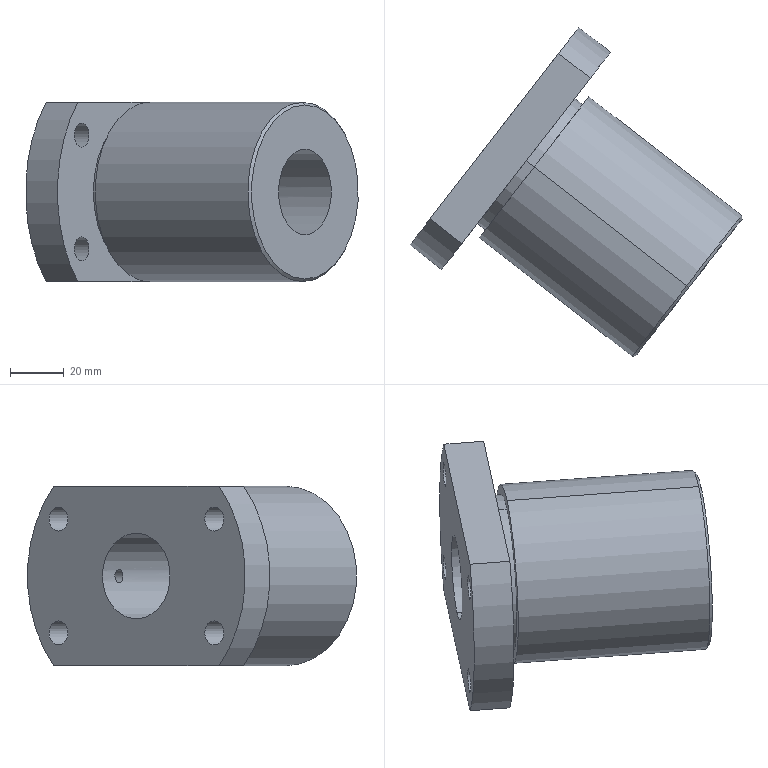Component | SolidWorks | MISUMI_BSSRK3210-800-F34-P20-1_NAT-2_MISUMI_BSSRK3210-800-F34-P20-1 | 1 solid | 26 faces | box 124.18 x 122.94 x 67 mm | volume 285610 mm3 | cylinder 18 | plane 6 | cone 2 | commonest cylinder face diameters 9 x8 4.917 x2 67 x2 59.3 x2 32 x2 103 x2
STEP:
#1=COLOUR_RGB('',0.7922,0.8196,0.9333);
#2=FILL_AREA_STYLE_COLOUR('',#1);
#3=FILL_AREA_STYLE('',(#2));
#4=SURFACE_STYLE_FILL_AREA(#3);
#5=SURFACE_SIDE_STYLE('',(#4));
#6=SURFACE_STYLE_USAGE(.BOTH.,#5);
#7=PRESENTATION_STYLE_ASSIGNMENT((#6));
#8=CARTESIAN_POINT('',(5.239,25.25,12.162));
#9=VERTEX_POINT('',#8);
#10=CARTESIAN_POINT('',(5.239,25.25,9.603));
#11=VERTEX_POINT('',#10);
#12=CARTESIAN_POINT('',(5.239,25.25,10.882));
#13=DIRECTION('',(0.7899,-0.6132,-0.));
#14=DIRECTION('',(0.,0.,-1.));
#15=AXIS2_PLACEMENT_3D('',#12,#13,#14);
#16=CIRCLE('',#15,1.28);
#17=EDGE_CURVE('',#9,#11,#16,.T.);
#18=ORIENTED_EDGE('',*,*,#17,.F.);
#19=CARTESIAN_POINT('',(5.208,25.274,12.201));
#20=VERTEX_POINT('',#19);
#21=CARTESIAN_POINT('',(5.239,25.25,12.162));
#22=DIRECTION('',(-0.5586,0.4336,0.7071));
#23=VECTOR('',#22,39.37);
#24=LINE('',#21,#23);
#25=EDGE_CURVE('',#9,#20,#24,.T.);
#26=ORIENTED_EDGE('',*,*,#25,.T.);
#27=CARTESIAN_POINT('',(5.208,25.274,9.563));
#28=VERTEX_POINT('',#27);
#29=CARTESIAN_POINT('',(5.208,25.274,10.882));
#30=DIRECTION('',(-0.7899,0.6132,0.));
#31=DIRECTION('',(0.,0.,-1.));
#32=AXIS2_PLACEMENT_3D('',#29,#30,#31);
#33=CIRCLE('',#32,1.319);
#34=EDGE_CURVE('',#28,#20,#33,.T.);
#35=ORIENTED_EDGE('',*,*,#34,.F.);
#36=CARTESIAN_POINT('',(5.239,25.25,9.603));
#37=DIRECTION('',(-0.5586,0.4336,-0.7071));
#38=VECTOR('',#37,39.37);
#39=LINE('',#36,#38);
#40=EDGE_CURVE('',#11,#28,#39,.T.);
#41=ORIENTED_EDGE('',*,*,#40,.F.);
#42=EDGE_LOOP('',(#18,#26,#35,#41));
#43=FACE_OUTER_BOUND('',#42,.T.);
#44=CARTESIAN_POINT('',(5.239,25.25,10.882));
#45=DIRECTION('',(-0.7899,0.6132,0.));
#46=DIRECTION('',(0.,0.,-1.));
#47=AXIS2_PLACEMENT_3D('',#44,#45,#46);
#48=CONICAL_SURFACE('',#47,1.28,0.7854);
#49=ADVANCED_FACE('',(#43),#48,.T.);
#50=CARTESIAN_POINT('',(3.071,27.721,10.979));
#51=VERTEX_POINT('',#50);
#52=CARTESIAN_POINT('',(3.071,27.721,10.786));
#53=VERTEX_POINT('',#52);
#54=CARTESIAN_POINT('',(3.071,27.721,10.979));
#55=CARTESIAN_POINT('',(3.081,27.713,10.979));
#56=CARTESIAN_POINT('',(3.091,27.706,10.977));
#57=CARTESIAN_POINT('',(3.105,27.696,10.969));
#58=CARTESIAN_POINT('',(3.11,27.693,10.966));
#59=CARTESIAN_POINT('',(3.119,27.687,10.959));
#60=CARTESIAN_POINT('',(3.123,27.684,10.955));
#61=CARTESIAN_POINT('',(3.131,27.68,10.946));
#62=CARTESIAN_POINT('',(3.134,27.677,10.941));
#63=CARTESIAN_POINT('',(3.14,27.674,10.931));
#64=CARTESIAN_POINT('',(3.143,27.672,10.925));
#65=CARTESIAN_POINT('',(3.147,27.67,10.914));
#66=CARTESIAN_POINT('',(3.149,27.669,10.907));
#67=CARTESIAN_POINT('',(3.151,27.668,10.895));
#68=CARTESIAN_POINT('',(3.152,27.667,10.889));
#69=CARTESIAN_POINT('',(3.152,27.667,10.876));
#70=CARTESIAN_POINT('',(3.151,27.668,10.87));
#71=CARTESIAN_POINT('',(3.149,27.669,10.857));
#72=CARTESIAN_POINT('',(3.147,27.67,10.851));
#73=CARTESIAN_POINT('',(3.143,27.672,10.839));
#74=CARTESIAN_POINT('',(3.141,27.674,10.834));
#75=CARTESIAN_POINT('',(3.134,27.677,10.823));
#76=CARTESIAN_POINT('',(3.131,27.68,10.818));
#77=CARTESIAN_POINT('',(3.119,27.687,10.805));
#78=CARTESIAN_POINT('',(3.11,27.692,10.798));
#79=CARTESIAN_POINT('',(3.096,27.702,10.791));
#80=CARTESIAN_POINT('',(3.091,27.706,10.789));
#81=CARTESIAN_POINT('',(3.081,27.713,10.786));
#82=CARTESIAN_POINT('',(3.076,27.717,10.786));
#83=CARTESIAN_POINT('',(3.071,27.721,10.786));
#84=B_SPLINE_CURVE_WITH_KNOTS('',3,(#54,#55,#56,#57,#58,#59,#60,#61,#62,#63,#64,#65,#66,#67,#68,#69,#70,#71,#72,#73,#74,#75,#76,#77,#78,#79,#80,#81,#82,#83),.UNSPECIFIED.,.F.,.F.,(4,2,2,2,2,2,2,2,2,2,2,2,2,2,4),(0.007698,0.00866,0.009141,0.009622,0.0101,0.01058,0.01106,0.01155,0.01203,0.01251,0.01299,0.01347,0.01443,0.01491,0.01539),.UNSPECIFIED.);
#85=EDGE_CURVE('',#51,#53,#84,.T.);
#86=ORIENTED_EDGE('',*,*,#85,.F.);
#87=CARTESIAN_POINT('',(3.931,28.829,10.979));
#88=VERTEX_POINT('',#87);
#89=CARTESIAN_POINT('',(3.932,28.831,10.979));
#90=DIRECTION('',(0.6132,0.7899,0.));
#91=VECTOR('',#90,39.37);
#92=LINE('',#89,#91);
#93=EDGE_CURVE('',#51,#88,#92,.T.);
#94=ORIENTED_EDGE('',*,*,#93,.T.);
#95=CARTESIAN_POINT('',(3.931,28.829,10.786));
#96=VERTEX_POINT('',#95);
#97=CARTESIAN_POINT('',(3.931,28.829,10.786));
#98=CARTESIAN_POINT('',(3.936,28.825,10.786));
#99=CARTESIAN_POINT('',(3.941,28.821,10.786));
#100=CARTESIAN_POINT('',(3.951,28.814,10.789));
#101=CARTESIAN_POINT('',(3.956,28.81,10.79));
#102=CARTESIAN_POINT('',(3.965,28.803,10.795));
#103=CARTESIAN_POINT('',(3.97,28.8,10.798));
#104=CARTESIAN_POINT('',(3.978,28.794,10.805));
#105=CARTESIAN_POINT('',(3.982,28.791,10.809));
#106=CARTESIAN_POINT('',(3.989,28.785,10.818));
#107=CARTESIAN_POINT('',(3.993,28.783,10.823));
#108=CARTESIAN_POINT('',(3.998,28.779,10.834));
#109=CARTESIAN_POINT('',(4.001,28.777,10.839));
#110=CARTESIAN_POINT('',(4.007,28.773,10.857));
#111=CARTESIAN_POINT('',(4.009,28.771,10.87));
#112=CARTESIAN_POINT('',(4.009,28.771,10.889));
#113=CARTESIAN_POINT('',(4.008,28.772,10.895));
#114=CARTESIAN_POINT('',(4.006,28.773,10.907));
#115=CARTESIAN_POINT('',(4.005,28.774,10.913));
#116=CARTESIAN_POINT('',(4.001,28.777,10.925));
#117=CARTESIAN_POINT('',(3.998,28.779,10.931));
#118=CARTESIAN_POINT('',(3.993,28.783,10.941));
#119=CARTESIAN_POINT('',(3.989,28.785,10.946));
#120=CARTESIAN_POINT('',(3.982,28.791,10.955));
#121=CARTESIAN_POINT('',(3.978,28.793,10.959));
#122=CARTESIAN_POINT('',(3.97,28.8,10.966));
#123=CARTESIAN_POINT('',(3.965,28.803,10.969));
#124=CARTESIAN_POINT('',(3.956,28.81,10.974));
#125=CARTESIAN_POINT('',(3.951,28.814,10.976));
#126=CARTESIAN_POINT('',(3.941,28.821,10.978));
#127=CARTESIAN_POINT('',(3.936,28.825,10.979));
#128=CARTESIAN_POINT('',(3.931,28.829,10.979));
#129=B_SPLINE_CURVE_WITH_KNOTS('',3,(#97,#98,#99,#100,#101,#102,#103,#104,#105,#106,#107,#108,#109,#110,#111,#112,#113,#114,#115,#116,#117,#118,#119,#120,#121,#122,#123,#124,#125,#126,#127,#128),.UNSPECIFIED.,.F.,.F.,(4,2,2,2,2,2,2,2,2,2,2,2,2,2,2,4),(0.,0.0004805,0.0009609,0.001441,0.001922,0.002402,0.002883,0.003844,0.004324,0.004805,0.005285,0.005766,0.006246,0.006727,0.007207,0.007687),.UNSPECIFIED.);
#130=EDGE_CURVE('',#96,#88,#129,.T.);
#131=ORIENTED_EDGE('',*,*,#130,.F.);
#132=CARTESIAN_POINT('',(3.932,28.831,10.786));
#133=DIRECTION('',(0.6132,0.7899,0.));
#134=VECTOR('',#133,39.37);
#135=LINE('',#132,#134);
#136=EDGE_CURVE('',#53,#96,#135,.T.);
#137=ORIENTED_EDGE('',*,*,#136,.F.);
#138=EDGE_LOOP('',(#86,#94,#131,#137));
#139=FACE_OUTER_BOUND('',#138,.T.);
#140=CARTESIAN_POINT('',(3.932,28.831,10.882));
#141=DIRECTION('',(0.6132,0.7899,0.));
#142=DIRECTION('',(0.,0.,-1.));
#143=AXIS2_PLACEMENT_3D('',#140,#141,#142);
#144=CYLINDRICAL_SURFACE('',#143,0.09679);
#145=ADVANCED_FACE('',(#139),#144,.F.);
#146=CARTESIAN_POINT('',(3.267,28.615,10.223));
#147=VERTEX_POINT('',#146);
#148=CARTESIAN_POINT('',(3.267,28.615,9.869));
#149=VERTEX_POINT('',#148);
#150=CARTESIAN_POINT('',(3.267,28.615,10.046));
#151=DIRECTION('',(-0.7899,0.6132,0.));
#152=DIRECTION('',(0.,0.,-1.));
#153=AXIS2_PLACEMENT_3D('',#150,#151,#152);
#154=CIRCLE('',#153,0.1772);
#155=EDGE_CURVE('',#147,#149,#154,.T.);
#156=ORIENTED_EDGE('',*,*,#155,.T.);
#157=CARTESIAN_POINT('',(3.733,28.253,9.869));
#158=VERTEX_POINT('',#157);
#159=CARTESIAN_POINT('',(3.267,28.615,9.869));
#160=DIRECTION('',(0.7899,-0.6132,-0.));
#161=VECTOR('',#160,39.37);
#162=LINE('',#159,#161);
#163=EDGE_CURVE('',#149,#158,#162,.T.);
#164=ORIENTED_EDGE('',*,*,#163,.T.);
#165=CARTESIAN_POINT('',(3.733,28.253,10.223));
#166=VERTEX_POINT('',#165);
#167=CARTESIAN_POINT('',(3.733,28.253,10.046));
#168=DIRECTION('',(-0.7899,0.6132,0.));
#169=DIRECTION('',(0.,0.,-1.));
#170=AXIS2_PLACEMENT_3D('',#167,#168,#169);
#171=CIRCLE('',#170,0.1772);
#172=EDGE_CURVE('',#166,#158,#171,.T.);
#173=ORIENTED_EDGE('',*,*,#172,.F.);
#174=CARTESIAN_POINT('',(3.267,28.615,10.223));
#175=DIRECTION('',(0.7899,-0.6132,-0.));
#176=VECTOR('',#175,39.37);
#177=LINE('',#174,#176);
#178=EDGE_CURVE('',#147,#166,#177,.T.);
#179=ORIENTED_EDGE('',*,*,#178,.F.);
#180=EDGE_LOOP('',(#156,#164,#173,#179));
#181=FACE_OUTER_BOUND('',#180,.T.);
#182=CARTESIAN_POINT('',(3.267,28.615,10.046));
#183=DIRECTION('',(0.7899,-0.6132,-0.));
#184=DIRECTION('',(-0.,-0.,1.));
#185=AXIS2_PLACEMENT_3D('',#182,#183,#184);
#186=CYLINDRICAL_SURFACE('',#185,0.1772);
#187=ADVANCED_FACE('',(#181),#186,.F.);
#188=CARTESIAN_POINT('',(3.267,28.615,11.896));
#189=VERTEX_POINT('',#188);
#190=CARTESIAN_POINT('',(3.267,28.615,11.542));
#191=VERTEX_POINT('',#190);
#192=CARTESIAN_POINT('',(3.267,28.615,11.719));
#193=DIRECTION('',(-0.7899,0.6132,0.));
#194=DIRECTION('',(0.,0.,-1.));
#195=AXIS2_PLACEMENT_3D('',#192,#193,#194);
#196=CIRCLE('',#195,0.1772);
#197=EDGE_CURVE('',#189,#191,#196,.T.);
#198=ORIENTED_EDGE('',*,*,#197,.T.);
#199=CARTESIAN_POINT('',(3.733,28.253,11.542));
#200=VERTEX_POINT('',#199);
#201=CARTESIAN_POINT('',(3.267,28.615,11.542));
#202=DIRECTION('',(0.7899,-0.6132,-0.));
#203=VECTOR('',#202,39.37);
#204=LINE('',#201,#203);
#205=EDGE_CURVE('',#191,#200,#204,.T.);
#206=ORIENTED_EDGE('',*,*,#205,.T.);
#207=CARTESIAN_POINT('',(3.733,28.253,11.896));
#208=VERTEX_POINT('',#207);
#209=CARTESIAN_POINT('',(3.733,28.253,11.719));
#210=DIRECTION('',(-0.7899,0.6132,0.));
#211=DIRECTION('',(0.,0.,-1.));
#212=AXIS2_PLACEMENT_3D('',#209,#210,#211);
#213=CIRCLE('',#212,0.1772);
#214=EDGE_CURVE('',#208,#200,#213,.T.);
#215=ORIENTED_EDGE('',*,*,#214,.F.);
#216=CARTESIAN_POINT('',(3.267,28.615,11.896));
#217=DIRECTION('',(0.7899,-0.6132,-0.));
#218=VECTOR('',#217,39.37);
#219=LINE('',#216,#218);
#220=EDGE_CURVE('',#189,#208,#219,.T.);
#221=ORIENTED_EDGE('',*,*,#220,.F.);
#222=EDGE_LOOP('',(#198,#206,#215,#221));
#223=FACE_OUTER_BOUND('',#222,.T.);
#224=CARTESIAN_POINT('',(3.267,28.615,11.719));
#225=DIRECTION('',(0.7899,-0.6132,-0.));
#226=DIRECTION('',(-0.,-0.,1.));
#227=AXIS2_PLACEMENT_3D('',#224,#225,#226);
#228=CYLINDRICAL_SURFACE('',#227,0.1772);
#229=ADVANCED_FACE('',(#223),#228,.F.);
#230=CARTESIAN_POINT('',(1.489,26.326,11.896));
#231=VERTEX_POINT('',#230);
#232=CARTESIAN_POINT('',(1.489,26.326,11.542));
#233=VERTEX_POINT('',#232);
#234=CARTESIAN_POINT('',(1.489,26.326,11.719));
#235=DIRECTION('',(-0.7899,0.6132,0.));
#236=DIRECTION('',(0.,0.,-1.));
#237=AXIS2_PLACEMENT_3D('',#234,#235,#236);
#238=CIRCLE('',#237,0.1772);
#239=EDGE_CURVE('',#231,#233,#238,.T.);
#240=ORIENTED_EDGE('',*,*,#239,.T.);
#241=CARTESIAN_POINT('',(1.956,25.964,11.542));
#242=VERTEX_POINT('',#241);
#243=CARTESIAN_POINT('',(1.489,26.326,11.542));
#244=DIRECTION('',(0.7899,-0.6132,-0.));
#245=VECTOR('',#244,39.37);
#246=LINE('',#243,#245);
#247=EDGE_CURVE('',#233,#242,#246,.T.);
#248=ORIENTED_EDGE('',*,*,#247,.T.);
#249=CARTESIAN_POINT('',(1.956,25.964,11.896));
#250=VERTEX_POINT('',#249);
#251=CARTESIAN_POINT('',(1.956,25.964,11.719));
#252=DIRECTION('',(-0.7899,0.6132,0.));
#253=DIRECTION('',(0.,0.,-1.));
#254=AXIS2_PLACEMENT_3D('',#251,#252,#253);
#255=CIRCLE('',#254,0.1772);
#256=EDGE_CURVE('',#250,#242,#255,.T.);
#257=ORIENTED_EDGE('',*,*,#256,.F.);
#258=CARTESIAN_POINT('',(1.489,26.326,11.896));
#259=DIRECTION('',(0.7899,-0.6132,-0.));
#260=VECTOR('',#259,39.37);
#261=LINE('',#258,#260);
#262=EDGE_CURVE('',#231,#250,#261,.T.);
#263=ORIENTED_EDGE('',*,*,#262,.F.);
#264=EDGE_LOOP('',(#240,#248,#257,#263));
#265=FACE_OUTER_BOUND('',#264,.T.);
#266=CARTESIAN_POINT('',(1.489,26.326,11.719));
#267=DIRECTION('',(0.7899,-0.6132,-0.));
#268=DIRECTION('',(-0.,-0.,1.));
#269=AXIS2_PLACEMENT_3D('',#266,#267,#268);
#270=CYLINDRICAL_SURFACE('',#269,0.1772);
#271=ADVANCED_FACE('',(#265),#270,.F.);
#272=CARTESIAN_POINT('',(1.489,26.326,10.223));
#273=VERTEX_POINT('',#272);
#274=CARTESIAN_POINT('',(1.489,26.326,9.869));
#275=VERTEX_POINT('',#274);
#276=CARTESIAN_POINT('',(1.489,26.326,10.046));
#277=DIRECTION('',(-0.7899,0.6132,0.));
#278=DIRECTION('',(0.,0.,-1.));
#279=AXIS2_PLACEMENT_3D('',#276,#277,#278);
#280=CIRCLE('',#279,0.1772);
#281=EDGE_CURVE('',#273,#275,#280,.T.);
#282=ORIENTED_EDGE('',*,*,#281,.T.);
#283=CARTESIAN_POINT('',(1.956,25.964,9.869));
#284=VERTEX_POINT('',#283);
#285=CARTESIAN_POINT('',(1.489,26.326,9.869));
#286=DIRECTION('',(0.7899,-0.6132,-0.));
#287=VECTOR('',#286,39.37);
#288=LINE('',#285,#287);
#289=EDGE_CURVE('',#275,#284,#288,.T.);
#290=ORIENTED_EDGE('',*,*,#289,.T.);
#291=CARTESIAN_POINT('',(1.956,25.964,10.223));
#292=VERTEX_POINT('',#291);
#293=CARTESIAN_POINT('',(1.956,25.964,10.046));
#294=DIRECTION('',(-0.7899,0.6132,0.));
#295=DIRECTION('',(0.,0.,-1.));
#296=AXIS2_PLACEMENT_3D('',#293,#294,#295);
#297=CIRCLE('',#296,0.1772);
#298=EDGE_CURVE('',#292,#284,#297,.T.);
#299=ORIENTED_EDGE('',*,*,#298,.F.);
#300=CARTESIAN_POINT('',(1.489,26.326,10.223));
#301=DIRECTION('',(0.7899,-0.6132,-0.));
#302=VECTOR('',#301,39.37);
#303=LINE('',#300,#302);
#304=EDGE_CURVE('',#273,#292,#303,.T.);
#305=ORIENTED_EDGE('',*,*,#304,.F.);
#306=EDGE_LOOP('',(#282,#290,#299,#305));
#307=FACE_OUTER_BOUND('',#306,.T.);
#308=CARTESIAN_POINT('',(1.489,26.326,10.046));
#309=DIRECTION('',(0.7899,-0.6132,-0.));
#310=DIRECTION('',(-0.,-0.,1.));
#311=AXIS2_PLACEMENT_3D('',#308,#309,#310);
#312=CYLINDRICAL_SURFACE('',#311,0.1772);
#313=ADVANCED_FACE('',(#307),#312,.F.);
#314=CARTESIAN_POINT('',(2.964,27.016,12.201));
#315=VERTEX_POINT('',#314);
#316=CARTESIAN_POINT('',(2.964,27.016,9.563));
#317=VERTEX_POINT('',#316);
#318=CARTESIAN_POINT('',(2.964,27.016,10.882));
#319=DIRECTION('',(0.7899,-0.6132,-0.));
#320=DIRECTION('',(-0.,-0.,1.));
#321=AXIS2_PLACEMENT_3D('',#318,#319,#320);
#322=CIRCLE('',#321,1.319);
#323=EDGE_CURVE('',#315,#317,#322,.T.);
#324=ORIENTED_EDGE('',*,*,#323,.T.);
#325=CARTESIAN_POINT('',(5.239,25.25,9.563));
#326=DIRECTION('',(0.7899,-0.6132,-0.));
#327=VECTOR('',#326,39.37);
#328=LINE('',#325,#327);
#329=EDGE_CURVE('',#317,#28,#328,.T.);
#330=ORIENTED_EDGE('',*,*,#329,.T.);
#331=ORIENTED_EDGE('',*,*,#34,.T.);
#332=CARTESIAN_POINT('',(5.239,25.25,12.201));
#333=DIRECTION('',(0.7899,-0.6132,-0.));
#334=VECTOR('',#333,39.37);
#335=LINE('',#332,#334);
#336=EDGE_CURVE('',#315,#20,#335,.T.);
#337=ORIENTED_EDGE('',*,*,#336,.F.);
#338=EDGE_LOOP('',(#324,#330,#331,#337));
#339=FACE_OUTER_BOUND('',#338,.T.);
#340=CARTESIAN_POINT('',(5.239,25.25,10.882));
#341=DIRECTION('',(0.7899,-0.6132,-0.));
#342=DIRECTION('',(-0.,-0.,1.));
#343=AXIS2_PLACEMENT_3D('',#340,#341,#342);
#344=CYLINDRICAL_SURFACE('',#343,1.319);
#345=ADVANCED_FACE('',(#339),#344,.T.);
#346=CARTESIAN_POINT('',(2.844,27.108,12.05));
#347=VERTEX_POINT('',#346);
#348=CARTESIAN_POINT('',(2.844,27.108,9.715));
#349=VERTEX_POINT('',#348);
#350=CARTESIAN_POINT('',(2.844,27.108,10.882));
#351=DIRECTION('',(0.7899,-0.6132,-0.));
#352=DIRECTION('',(-0.,-0.,1.));
#353=AXIS2_PLACEMENT_3D('',#350,#351,#352);
#354=CIRCLE('',#353,1.167);
#355=EDGE_CURVE('',#347,#349,#354,.T.);
#356=ORIENTED_EDGE('',*,*,#355,.T.);
#357=CARTESIAN_POINT('',(2.964,27.016,9.715));
#358=VERTEX_POINT('',#357);
#359=CARTESIAN_POINT('',(5.239,25.25,9.715));
#360=DIRECTION('',(0.7899,-0.6132,-0.));
#361=VECTOR('',#360,39.37);
#362=LINE('',#359,#361);
#363=EDGE_CURVE('',#349,#358,#362,.T.);
#364=ORIENTED_EDGE('',*,*,#363,.T.);
#365=CARTESIAN_POINT('',(2.964,27.016,12.05));
#366=VERTEX_POINT('',#365);
#367=CARTESIAN_POINT('',(2.964,27.016,10.882));
#368=DIRECTION('',(0.7899,-0.6132,-0.));
#369=DIRECTION('',(-0.,-0.,1.));
#370=AXIS2_PLACEMENT_3D('',#367,#368,#369);
#371=CIRCLE('',#370,1.167);
#372=EDGE_CURVE('',#366,#358,#371,.T.);
#373=ORIENTED_EDGE('',*,*,#372,.F.);
#374=CARTESIAN_POINT('',(5.239,25.25,12.05));
#375=DIRECTION('',(0.7899,-0.6132,-0.));
#376=VECTOR('',#375,39.37);
#377=LINE('',#374,#376);
#378=EDGE_CURVE('',#347,#366,#377,.T.);
#379=ORIENTED_EDGE('',*,*,#378,.F.);
#380=EDGE_LOOP('',(#356,#364,#373,#379));
#381=FACE_OUTER_BOUND('',#380,.T.);
#382=CARTESIAN_POINT('',(5.239,25.25,10.882));
#383=DIRECTION('',(0.7899,-0.6132,-0.));
#384=DIRECTION('',(-0.,-0.,1.));
#385=AXIS2_PLACEMENT_3D('',#382,#383,#384);
#386=CYLINDRICAL_SURFACE('',#385,1.167);
#387=ADVANCED_FACE('',(#381),#386,.T.);
#388=CARTESIAN_POINT('',(3.071,27.721,10.786));
#389=CARTESIAN_POINT('',(3.066,27.725,10.786));
#390=CARTESIAN_POINT('',(3.061,27.729,10.786));
#391=CARTESIAN_POINT('',(3.051,27.737,10.789));
#392=CARTESIAN_POINT('',(3.046,27.741,10.79));
#393=CARTESIAN_POINT('',(3.038,27.748,10.795));
#394=CARTESIAN_POINT('',(3.033,27.752,10.798));
#395=CARTESIAN_POINT('',(3.026,27.759,10.805));
#396=CARTESIAN_POINT('',(3.022,27.763,10.809));
#397=CARTESIAN_POINT('',(3.012,27.772,10.823));
#398=CARTESIAN_POINT('',(3.007,27.777,10.834));
#399=CARTESIAN_POINT('',(3.002,27.783,10.851));
#400=CARTESIAN_POINT('',(3.001,27.784,10.857));
#401=CARTESIAN_POINT('',(2.999,27.786,10.87));
#402=CARTESIAN_POINT('',(2.999,27.786,10.876));
#403=CARTESIAN_POINT('',(2.999,27.786,10.889));
#404=CARTESIAN_POINT('',(2.999,27.786,10.895));
#405=CARTESIAN_POINT('',(3.001,27.784,10.907));
#406=CARTESIAN_POINT('',(3.002,27.783,10.914));
#407=CARTESIAN_POINT('',(3.006,27.779,10.925));
#408=CARTESIAN_POINT('',(3.008,27.777,10.931));
#409=CARTESIAN_POINT('',(3.013,27.772,10.941));
#410=CARTESIAN_POINT('',(3.016,27.769,10.946));
#411=CARTESIAN_POINT('',(3.022,27.763,10.955));
#412=CARTESIAN_POINT('',(3.026,27.759,10.959));
#413=CARTESIAN_POINT('',(3.033,27.752,10.966));
#414=CARTESIAN_POINT('',(3.038,27.748,10.969));
#415=CARTESIAN_POINT('',(3.046,27.741,10.974));
#416=CARTESIAN_POINT('',(3.051,27.737,10.976));
#417=CARTESIAN_POINT('',(3.061,27.729,10.978));
#418=CARTESIAN_POINT('',(3.066,27.725,10.979));
#419=CARTESIAN_POINT('',(3.071,27.721,10.979));
#420=B_SPLINE_CURVE_WITH_KNOTS('',3,(#388,#389,#390,#391,#392,#393,#394,#395,#396,#397,#398,#399,#400,#401,#402,#403,#404,#405,#406,#407,#408,#409,#410,#411,#412,#413,#414,#415,#416,#417,#418,#419),.UNSPECIFIED.,.F.,.F.,(4,2,2,2,2,2,2,2,2,2,2,2,2,2,2,4),(0.,0.0004811,0.0009622,0.001443,0.001924,0.002887,0.003368,0.003849,0.00433,0.004811,0.005292,0.005773,0.006254,0.006736,0.007217,0.007698),.UNSPECIFIED.);
#421=EDGE_CURVE('',#53,#51,#420,.T.);
#422=ORIENTED_EDGE('',*,*,#421,.T.);
#423=ORIENTED_EDGE('',*,*,#85,.T.);
#424=EDGE_LOOP('',(#422,#423));
#425=FACE_BOUND('',#424,.T.);
#426=CARTESIAN_POINT('',(2.378,27.471,10.252));
#427=VERTEX_POINT('',#426);
#428=CARTESIAN_POINT('',(2.378,27.471,11.512));
#429=VERTEX_POINT('',#428);
#430=CARTESIAN_POINT('',(2.378,27.471,10.882));
#431=DIRECTION('',(0.7899,-0.6132,-0.));
#432=DIRECTION('',(-0.,-0.,1.));
#433=AXIS2_PLACEMENT_3D('',#430,#431,#432);
#434=CIRCLE('',#433,0.6299);
#435=EDGE_CURVE('',#427,#429,#434,.T.);
#436=ORIENTED_EDGE('',*,*,#435,.F.);
#437=CARTESIAN_POINT('',(5.239,25.25,10.252));
#438=VERTEX_POINT('',#437);
#439=CARTESIAN_POINT('',(5.239,25.25,10.252));
#440=DIRECTION('',(0.7899,-0.6132,-0.));
#441=VECTOR('',#440,39.37);
#442=LINE('',#439,#441);
#443=EDGE_CURVE('',#427,#438,#442,.T.);
#444=ORIENTED_EDGE('',*,*,#443,.T.);
#445=CARTESIAN_POINT('',(5.239,25.25,11.512));
#446=VERTEX_POINT('',#445);
#447=CARTESIAN_POINT('',(5.239,25.25,10.882));
#448=DIRECTION('',(0.7899,-0.6132,-0.));
#449=DIRECTION('',(-0.,-0.,1.));
#450=AXIS2_PLACEMENT_3D('',#447,#448,#449);
#451=CIRCLE('',#450,0.6299);
#452=EDGE_CURVE('',#438,#446,#451,.T.);
#453=ORIENTED_EDGE('',*,*,#452,.T.);
#454=CARTESIAN_POINT('',(5.239,25.25,11.512));
#455=DIRECTION('',(0.7899,-0.6132,-0.));
#456=VECTOR('',#455,39.37);
#457=LINE('',#454,#456);
#458=EDGE_CURVE('',#429,#446,#457,.T.);
#459=ORIENTED_EDGE('',*,*,#458,.F.);
#460=EDGE_LOOP('',(#436,#444,#453,#459));
#461=FACE_OUTER_BOUND('',#460,.T.);
#462=CARTESIAN_POINT('',(5.239,25.25,10.882));
#463=DIRECTION('',(0.7899,-0.6132,-0.));
#464=DIRECTION('',(-0.,-0.,1.));
#465=AXIS2_PLACEMENT_3D('',#462,#463,#464);
#466=CYLINDRICAL_SURFACE('',#465,0.6299);
#467=ADVANCED_FACE('',(#425,#461),#466,.F.);
#468=CARTESIAN_POINT('',(2.378,27.471,10.882));
#469=DIRECTION('',(0.7899,-0.6132,-0.));
#470=DIRECTION('',(-0.,-0.,1.));
#471=AXIS2_PLACEMENT_3D('',#468,#469,#470);
#472=CIRCLE('',#471,0.6299);
#473=EDGE_CURVE('',#429,#427,#472,.T.);
#474=ORIENTED_EDGE('',*,*,#473,.T.);
#475=ORIENTED_EDGE('',*,*,#435,.T.);
#476=EDGE_LOOP('',(#474,#475));
#477=FACE_BOUND('',#476,.T.);
#478=CARTESIAN_POINT('',(3.322,28.687,12.201));
#479=VERTEX_POINT('',#478);
#480=CARTESIAN_POINT('',(1.434,26.254,12.201));
#481=VERTEX_POINT('',#480);
#482=CARTESIAN_POINT('',(1.434,26.254,12.201));
#483=DIRECTION('',(-0.6132,-0.7899,-0.));
#484=VECTOR('',#483,39.37);
#485=LINE('',#482,#484);
#486=EDGE_CURVE('',#479,#481,#485,.T.);
#487=ORIENTED_EDGE('',*,*,#486,.F.);
#488=CARTESIAN_POINT('',(3.322,28.687,9.563));
#489=VERTEX_POINT('',#488);
#490=CARTESIAN_POINT('',(2.378,27.471,10.882));
#491=DIRECTION('',(0.7899,-0.6132,-0.));
#492=DIRECTION('',(-0.,-0.,1.));
#493=AXIS2_PLACEMENT_3D('',#490,#491,#492);
#494=CIRCLE('',#493,2.028);
#495=EDGE_CURVE('',#489,#479,#494,.T.);
#496=ORIENTED_EDGE('',*,*,#495,.F.);
#497=CARTESIAN_POINT('',(1.434,26.254,9.563));
#498=VERTEX_POINT('',#497);
#499=CARTESIAN_POINT('',(1.434,26.254,9.563));
#500=DIRECTION('',(0.6132,0.7899,0.));
#501=VECTOR('',#500,39.37);
#502=LINE('',#499,#501);
#503=EDGE_CURVE('',#498,#489,#502,.T.);
#504=ORIENTED_EDGE('',*,*,#503,.F.);
#505=CARTESIAN_POINT('',(2.378,27.471,10.882));
#506=DIRECTION('',(0.7899,-0.6132,-0.));
#507=DIRECTION('',(-0.,-0.,1.));
#508=AXIS2_PLACEMENT_3D('',#505,#506,#507);
#509=CIRCLE('',#508,2.028);
#510=EDGE_CURVE('',#481,#498,#509,.T.);
#511=ORIENTED_EDGE('',*,*,#510,.F.);
#512=EDGE_LOOP('',(#487,#496,#504,#511));
#513=FACE_OUTER_BOUND('',#512,.T.);
#514=ORIENTED_EDGE('',*,*,#281,.F.);
#515=CARTESIAN_POINT('',(1.489,26.326,10.046));
#516=DIRECTION('',(-0.7899,0.6132,0.));
#517=DIRECTION('',(0.,0.,-1.));
#518=AXIS2_PLACEMENT_3D('',#515,#516,#517);
#519=CIRCLE('',#518,0.1772);
#520=EDGE_CURVE('',#275,#273,#519,.T.);
#521=ORIENTED_EDGE('',*,*,#520,.F.);
#522=EDGE_LOOP('',(#514,#521));
#523=FACE_BOUND('',#522,.T.);
#524=ORIENTED_EDGE('',*,*,#239,.F.);
#525=CARTESIAN_POINT('',(1.489,26.326,11.719));
#526=DIRECTION('',(-0.7899,0.6132,0.));
#527=DIRECTION('',(0.,0.,-1.));
#528=AXIS2_PLACEMENT_3D('',#525,#526,#527);
#529=CIRCLE('',#528,0.1772);
#530=EDGE_CURVE('',#233,#231,#529,.T.);
#531=ORIENTED_EDGE('',*,*,#530,.F.);
#532=EDGE_LOOP('',(#524,#531));
#533=FACE_BOUND('',#532,.T.);
#534=ORIENTED_EDGE('',*,*,#197,.F.);
#535=CARTESIAN_POINT('',(3.267,28.615,11.719));
#536=DIRECTION('',(-0.7899,0.6132,0.));
#537=DIRECTION('',(0.,0.,-1.));
#538=AXIS2_PLACEMENT_3D('',#535,#536,#537);
#539=CIRCLE('',#538,0.1772);
#540=EDGE_CURVE('',#191,#189,#539,.T.);
#541=ORIENTED_EDGE('',*,*,#540,.F.);
#542=EDGE_LOOP('',(#534,#541));
#543=FACE_BOUND('',#542,.T.);
#544=ORIENTED_EDGE('',*,*,#155,.F.);
#545=CARTESIAN_POINT('',(3.267,28.615,10.046));
#546=DIRECTION('',(-0.7899,0.6132,0.));
#547=DIRECTION('',(0.,0.,-1.));
#548=AXIS2_PLACEMENT_3D('',#545,#546,#547);
#549=CIRCLE('',#548,0.1772);
#550=EDGE_CURVE('',#149,#147,#549,.T.);
#551=ORIENTED_EDGE('',*,*,#550,.F.);
#552=EDGE_LOOP('',(#544,#551));
#553=FACE_BOUND('',#552,.T.);
#554=CARTESIAN_POINT('',(1.992,26.973,10.882));
#555=DIRECTION('',(0.7899,-0.6132,-0.));
#556=DIRECTION('',(-0.,-0.,1.));
#557=AXIS2_PLACEMENT_3D('',#554,#555,#556);
#558=PLANE('',#557);
#559=ADVANCED_FACE('',(#477,#513,#523,#533,#543,#553),#558,.F.);
#560=ORIENTED_EDGE('',*,*,#355,.F.);
#561=CARTESIAN_POINT('',(2.844,27.108,10.882));
#562=DIRECTION('',(0.7899,-0.6132,-0.));
#563=DIRECTION('',(-0.,-0.,1.));
#564=AXIS2_PLACEMENT_3D('',#561,#562,#563);
#565=CIRCLE('',#564,1.167);
#566=EDGE_CURVE('',#349,#347,#565,.T.);
#567=ORIENTED_EDGE('',*,*,#566,.F.);
#568=EDGE_LOOP('',(#560,#567));
#569=FACE_BOUND('',#568,.T.);
#570=CARTESIAN_POINT('',(3.789,28.325,12.201));
#571=VERTEX_POINT('',#570);
#572=CARTESIAN_POINT('',(1.9,25.892,12.201));
#573=VERTEX_POINT('',#572);
#574=CARTESIAN_POINT('',(1.9,25.892,12.201));
#575=DIRECTION('',(-0.6132,-0.7899,-0.));
#576=VECTOR('',#575,39.37);
#577=LINE('',#574,#576);
#578=EDGE_CURVE('',#571,#573,#577,.T.);
#579=ORIENTED_EDGE('',*,*,#578,.T.);
#580=CARTESIAN_POINT('',(1.9,25.892,9.563));
#581=VERTEX_POINT('',#580);
#582=CARTESIAN_POINT('',(2.844,27.108,10.882));
#583=DIRECTION('',(0.7899,-0.6132,-0.));
#584=DIRECTION('',(-0.,-0.,1.));
#585=AXIS2_PLACEMENT_3D('',#582,#583,#584);
#586=CIRCLE('',#585,2.028);
#587=EDGE_CURVE('',#573,#581,#586,.T.);
#588=ORIENTED_EDGE('',*,*,#587,.T.);
#589=CARTESIAN_POINT('',(3.789,28.325,9.563));
#590=VERTEX_POINT('',#589);
#591=CARTESIAN_POINT('',(1.9,25.892,9.563));
#592=DIRECTION('',(0.6132,0.7899,0.));
#593=VECTOR('',#592,39.37);
#594=LINE('',#591,#593);
#595=EDGE_CURVE('',#581,#590,#594,.T.);
#596=ORIENTED_EDGE('',*,*,#595,.T.);
#597=CARTESIAN_POINT('',(2.844,27.108,10.882));
#598=DIRECTION('',(0.7899,-0.6132,-0.));
#599=DIRECTION('',(-0.,-0.,1.));
#600=AXIS2_PLACEMENT_3D('',#597,#598,#599);
#601=CIRCLE('',#600,2.028);
#602=EDGE_CURVE('',#590,#571,#601,.T.);
#603=ORIENTED_EDGE('',*,*,#602,.T.);
#604=EDGE_LOOP('',(#579,#588,#596,#603));
#605=FACE_OUTER_BOUND('',#604,.T.);
#606=ORIENTED_EDGE('',*,*,#298,.T.);
#607=CARTESIAN_POINT('',(1.956,25.964,10.046));
#608=DIRECTION('',(-0.7899,0.6132,0.));
#609=DIRECTION('',(0.,0.,-1.));
#610=AXIS2_PLACEMENT_3D('',#607,#608,#609);
#611=CIRCLE('',#610,0.1772);
#612=EDGE_CURVE('',#284,#292,#611,.T.);
#613=ORIENTED_EDGE('',*,*,#612,.T.);
#614=EDGE_LOOP('',(#606,#613));
#615=FACE_BOUND('',#614,.T.);
#616=ORIENTED_EDGE('',*,*,#256,.T.);
#617=CARTESIAN_POINT('',(1.956,25.964,11.719));
#618=DIRECTION('',(-0.7899,0.6132,0.));
#619=DIRECTION('',(0.,0.,-1.));
#620=AXIS2_PLACEMENT_3D('',#617,#618,#619);
#621=CIRCLE('',#620,0.1772);
#622=EDGE_CURVE('',#242,#250,#621,.T.);
#623=ORIENTED_EDGE('',*,*,#622,.T.);
#624=EDGE_LOOP('',(#616,#623));
#625=FACE_BOUND('',#624,.T.);
#626=ORIENTED_EDGE('',*,*,#214,.T.);
#627=CARTESIAN_POINT('',(3.733,28.253,11.719));
#628=DIRECTION('',(-0.7899,0.6132,0.));
#629=DIRECTION('',(0.,0.,-1.));
#630=AXIS2_PLACEMENT_3D('',#627,#628,#629);
#631=CIRCLE('',#630,0.1772);
#632=EDGE_CURVE('',#200,#208,#631,.T.);
#633=ORIENTED_EDGE('',*,*,#632,.T.);
#634=EDGE_LOOP('',(#626,#633));
#635=FACE_BOUND('',#634,.T.);
#636=ORIENTED_EDGE('',*,*,#172,.T.);
#637=CARTESIAN_POINT('',(3.733,28.253,10.046));
#638=DIRECTION('',(-0.7899,0.6132,0.));
#639=DIRECTION('',(0.,0.,-1.));
#640=AXIS2_PLACEMENT_3D('',#637,#638,#639);
#641=CIRCLE('',#640,0.1772);
#642=EDGE_CURVE('',#158,#166,#641,.T.);
#643=ORIENTED_EDGE('',*,*,#642,.T.);
#644=EDGE_LOOP('',(#636,#643));
#645=FACE_BOUND('',#644,.T.);
#646=CARTESIAN_POINT('',(1.601,25.507,10.882));
#647=DIRECTION('',(-0.7899,0.6132,0.));
#648=DIRECTION('',(0.,0.,-1.));
#649=AXIS2_PLACEMENT_3D('',#646,#647,#648);
#650=PLANE('',#649);
#651=ADVANCED_FACE('',(#569,#605,#615,#625,#635,#645),#650,.F.);
#652=CARTESIAN_POINT('',(1.434,26.254,12.201));
#653=DIRECTION('',(0.7899,-0.6132,-0.));
#654=VECTOR('',#653,39.37);
#655=LINE('',#652,#654);
#656=EDGE_CURVE('',#481,#573,#655,.T.);
#657=ORIENTED_EDGE('',*,*,#656,.F.);
#658=ORIENTED_EDGE('',*,*,#510,.T.);
#659=CARTESIAN_POINT('',(1.434,26.254,9.563));
#660=DIRECTION('',(0.7899,-0.6132,-0.));
#661=VECTOR('',#660,39.37);
#662=LINE('',#659,#661);
#663=EDGE_CURVE('',#498,#581,#662,.T.);
#664=ORIENTED_EDGE('',*,*,#663,.T.);
#665=ORIENTED_EDGE('',*,*,#587,.F.);
#666=EDGE_LOOP('',(#657,#658,#664,#665));
#667=FACE_OUTER_BOUND('',#666,.T.);
#668=CARTESIAN_POINT('',(5.239,25.25,10.882));
#669=DIRECTION('',(0.7899,-0.6132,-0.));
#670=DIRECTION('',(-0.,-0.,1.));
#671=AXIS2_PLACEMENT_3D('',#668,#669,#670);
#672=CYLINDRICAL_SURFACE('',#671,2.028);
#673=ADVANCED_FACE('',(#667),#672,.T.);
#674=ORIENTED_EDGE('',*,*,#130,.T.);
#675=CARTESIAN_POINT('',(3.931,28.829,10.979));
#676=CARTESIAN_POINT('',(3.926,28.833,10.979));
#677=CARTESIAN_POINT('',(3.921,28.837,10.979));
#678=CARTESIAN_POINT('',(3.911,28.844,10.976));
#679=CARTESIAN_POINT('',(3.906,28.848,10.974));
#680=CARTESIAN_POINT('',(3.893,28.859,10.967));
#681=CARTESIAN_POINT('',(3.884,28.866,10.96));
#682=CARTESIAN_POINT('',(3.874,28.875,10.946));
#683=CARTESIAN_POINT('',(3.871,28.877,10.941));
#684=CARTESIAN_POINT('',(3.866,28.882,10.931));
#685=CARTESIAN_POINT('',(3.863,28.884,10.925));
#686=CARTESIAN_POINT('',(3.86,28.887,10.914));
#687=CARTESIAN_POINT('',(3.858,28.888,10.907));
#688=CARTESIAN_POINT('',(3.856,28.89,10.895));
#689=CARTESIAN_POINT('',(3.856,28.89,10.889));
#690=CARTESIAN_POINT('',(3.856,28.89,10.876));
#691=CARTESIAN_POINT('',(3.856,28.89,10.87));
#692=CARTESIAN_POINT('',(3.858,28.888,10.857));
#693=CARTESIAN_POINT('',(3.86,28.887,10.851));
#694=CARTESIAN_POINT('',(3.863,28.884,10.839));
#695=CARTESIAN_POINT('',(3.866,28.882,10.834));
#696=CARTESIAN_POINT('',(3.871,28.877,10.823));
#697=CARTESIAN_POINT('',(3.874,28.875,10.818));
#698=CARTESIAN_POINT('',(3.881,28.869,10.809));
#699=CARTESIAN_POINT('',(3.885,28.866,10.805));
#700=CARTESIAN_POINT('',(3.893,28.859,10.798));
#701=CARTESIAN_POINT('',(3.897,28.856,10.795));
#702=CARTESIAN_POINT('',(3.911,28.845,10.788));
#703=CARTESIAN_POINT('',(3.921,28.837,10.786));
#704=CARTESIAN_POINT('',(3.931,28.829,10.786));
#705=B_SPLINE_CURVE_WITH_KNOTS('',3,(#675,#676,#677,#678,#679,#680,#681,#682,#683,#684,#685,#686,#687,#688,#689,#690,#691,#692,#693,#694,#695,#696,#697,#698,#699,#700,#701,#702,#703,#704),.UNSPECIFIED.,.F.,.F.,(4,2,2,2,2,2,2,2,2,2,2,2,2,2,4),(0.007687,0.008168,0.008648,0.009609,0.01009,0.01057,0.01105,0.01153,0.01201,0.01249,0.01297,0.01345,0.01393,0.01441,0.01537),.UNSPECIFIED.);
#706=EDGE_CURVE('',#88,#96,#705,.T.);
#707=ORIENTED_EDGE('',*,*,#706,.T.);
#708=EDGE_LOOP('',(#674,#707));
#709=FACE_BOUND('',#708,.T.);
#710=CARTESIAN_POINT('',(3.322,28.687,12.201));
#711=DIRECTION('',(0.7899,-0.6132,-0.));
#712=VECTOR('',#711,39.37);
#713=LINE('',#710,#712);
#714=EDGE_CURVE('',#479,#571,#713,.T.);
#715=ORIENTED_EDGE('',*,*,#714,.T.);
#716=ORIENTED_EDGE('',*,*,#602,.F.);
#717=CARTESIAN_POINT('',(3.322,28.687,9.563));
#718=DIRECTION('',(0.7899,-0.6132,-0.));
#719=VECTOR('',#718,39.37);
#720=LINE('',#717,#719);
#721=EDGE_CURVE('',#489,#590,#720,.T.);
#722=ORIENTED_EDGE('',*,*,#721,.F.);
#723=ORIENTED_EDGE('',*,*,#495,.T.);
#724=EDGE_LOOP('',(#715,#716,#722,#723));
#725=FACE_OUTER_BOUND('',#724,.T.);
#726=CARTESIAN_POINT('',(5.239,25.25,10.882));
#727=DIRECTION('',(0.7899,-0.6132,-0.));
#728=DIRECTION('',(-0.,-0.,1.));
#729=AXIS2_PLACEMENT_3D('',#726,#727,#728);
#730=CYLINDRICAL_SURFACE('',#729,2.028);
#731=ADVANCED_FACE('',(#709,#725),#730,.T.);
#732=ORIENTED_EDGE('',*,*,#443,.F.);
#733=ORIENTED_EDGE('',*,*,#473,.F.);
#734=ORIENTED_EDGE('',*,*,#458,.T.);
#735=CARTESIAN_POINT('',(5.239,25.25,10.882));
#736=DIRECTION('',(0.7899,-0.6132,-0.));
#737=DIRECTION('',(-0.,-0.,1.));
#738=AXIS2_PLACEMENT_3D('',#735,#736,#737);
#739=CIRCLE('',#738,0.6299);
#740=EDGE_CURVE('',#446,#438,#739,.T.);
#741=ORIENTED_EDGE('',*,*,#740,.T.);
#742=EDGE_LOOP('',(#732,#733,#734,#741));
#743=FACE_OUTER_BOUND('',#742,.T.);
#744=CARTESIAN_POINT('',(5.239,25.25,10.882));
#745=DIRECTION('',(0.7899,-0.6132,-0.));
#746=DIRECTION('',(-0.,-0.,1.));
#747=AXIS2_PLACEMENT_3D('',#744,#745,#746);
#748=CYLINDRICAL_SURFACE('',#747,0.6299);
#749=ADVANCED_FACE('',(#743),#748,.F.);
#750=ORIENTED_EDGE('',*,*,#363,.F.);
#751=ORIENTED_EDGE('',*,*,#566,.T.);
#752=ORIENTED_EDGE('',*,*,#378,.T.);
#753=CARTESIAN_POINT('',(2.964,27.016,10.882));
#754=DIRECTION('',(0.7899,-0.6132,-0.));
#755=DIRECTION('',(-0.,-0.,1.));
#756=AXIS2_PLACEMENT_3D('',#753,#754,#755);
#757=CIRCLE('',#756,1.167);
#758=EDGE_CURVE('',#358,#366,#757,.T.);
#759=ORIENTED_EDGE('',*,*,#758,.F.);
#760=EDGE_LOOP('',(#750,#751,#752,#759));
#761=FACE_OUTER_BOUND('',#760,.T.);
#762=CARTESIAN_POINT('',(5.239,25.25,10.882));
#763=DIRECTION('',(0.7899,-0.6132,-0.));
#764=DIRECTION('',(-0.,-0.,1.));
#765=AXIS2_PLACEMENT_3D('',#762,#763,#764);
#766=CYLINDRICAL_SURFACE('',#765,1.167);
#767=ADVANCED_FACE('',(#761),#766,.T.);
#768=ORIENTED_EDGE('',*,*,#323,.F.);
#769=CARTESIAN_POINT('',(2.964,27.016,10.882));
#770=DIRECTION('',(0.7899,-0.6132,-0.));
#771=DIRECTION('',(-0.,-0.,1.));
#772=AXIS2_PLACEMENT_3D('',#769,#770,#771);
#773=CIRCLE('',#772,1.319);
#774=EDGE_CURVE('',#317,#315,#773,.T.);
#775=ORIENTED_EDGE('',*,*,#774,.F.);
#776=EDGE_LOOP('',(#768,#775));
#777=FACE_OUTER_BOUND('',#776,.T.);
#778=ORIENTED_EDGE('',*,*,#372,.T.);
#779=ORIENTED_EDGE('',*,*,#758,.T.);
#780=EDGE_LOOP('',(#778,#779));
#781=FACE_BOUND('',#780,.T.);
#782=CARTESIAN_POINT('',(2.248,26.093,10.882));
#783=DIRECTION('',(0.7899,-0.6132,-0.));
#784=DIRECTION('',(-0.,-0.,1.));
#785=AXIS2_PLACEMENT_3D('',#782,#783,#784);
#786=PLANE('',#785);
#787=ADVANCED_FACE('',(#777,#781),#786,.F.);
#788=ORIENTED_EDGE('',*,*,#329,.F.);
#789=ORIENTED_EDGE('',*,*,#774,.T.);
#790=ORIENTED_EDGE('',*,*,#336,.T.);
#791=CARTESIAN_POINT('',(5.208,25.274,10.882));
#792=DIRECTION('',(-0.7899,0.6132,0.));
#793=DIRECTION('',(0.,0.,-1.));
#794=AXIS2_PLACEMENT_3D('',#791,#792,#793);
#795=CIRCLE('',#794,1.319);
#796=EDGE_CURVE('',#20,#28,#795,.T.);
#797=ORIENTED_EDGE('',*,*,#796,.T.);
#798=EDGE_LOOP('',(#788,#789,#790,#797));
#799=FACE_OUTER_BOUND('',#798,.T.);
#800=CARTESIAN_POINT('',(5.239,25.25,10.882));
#801=DIRECTION('',(0.7899,-0.6132,-0.));
#802=DIRECTION('',(-0.,-0.,1.));
#803=AXIS2_PLACEMENT_3D('',#800,#801,#802);
#804=CYLINDRICAL_SURFACE('',#803,1.319);
#805=ADVANCED_FACE('',(#799),#804,.T.);
#806=CARTESIAN_POINT('',(5.239,25.25,10.882));
#807=DIRECTION('',(0.7899,-0.6132,-0.));
#808=DIRECTION('',(0.,0.,-1.));
#809=AXIS2_PLACEMENT_3D('',#806,#807,#808);
#810=CIRCLE('',#809,1.28);
#811=EDGE_CURVE('',#11,#9,#810,.T.);
#812=ORIENTED_EDGE('',*,*,#811,.T.);
#813=ORIENTED_EDGE('',*,*,#17,.T.);
#814=EDGE_LOOP('',(#812,#813));
#815=FACE_OUTER_BOUND('',#814,.T.);
#816=ORIENTED_EDGE('',*,*,#740,.F.);
#817=ORIENTED_EDGE('',*,*,#452,.F.);
#818=EDGE_LOOP('',(#816,#817));
#819=FACE_BOUND('',#818,.T.);
#820=CARTESIAN_POINT('',(4.43,24.208,10.882));
#821=DIRECTION('',(-0.7899,0.6132,0.));
#822=DIRECTION('',(0.,0.,-1.));
#823=AXIS2_PLACEMENT_3D('',#820,#821,#822);
#824=PLANE('',#823);
#825=ADVANCED_FACE('',(#815,#819),#824,.F.);
#826=ORIENTED_EDGE('',*,*,#595,.F.);
#827=ORIENTED_EDGE('',*,*,#663,.F.);
#828=ORIENTED_EDGE('',*,*,#503,.T.);
#829=ORIENTED_EDGE('',*,*,#721,.T.);
#830=EDGE_LOOP('',(#826,#827,#828,#829));
#831=FACE_OUTER_BOUND('',#830,.T.);
#832=CARTESIAN_POINT('',(1.434,26.254,9.563));
#833=DIRECTION('',(0.,0.,-1.));
#834=DIRECTION('',(0.7899,-0.6132,-0.));
#835=AXIS2_PLACEMENT_3D('',#832,#833,#834);
#836=PLANE('',#835);
#837=ADVANCED_FACE('',(#831),#836,.T.);
#838=ORIENTED_EDGE('',*,*,#578,.F.);
#839=ORIENTED_EDGE('',*,*,#714,.F.);
#840=ORIENTED_EDGE('',*,*,#486,.T.);
#841=ORIENTED_EDGE('',*,*,#656,.T.);
#842=EDGE_LOOP('',(#838,#839,#840,#841));
#843=FACE_OUTER_BOUND('',#842,.T.);
#844=CARTESIAN_POINT('',(1.434,26.254,12.201));
#845=DIRECTION('',(-0.,-0.,1.));
#846=DIRECTION('',(-0.7899,0.6132,0.));
#847=AXIS2_PLACEMENT_3D('',#844,#845,#846);
#848=PLANE('',#847);
#849=ADVANCED_FACE('',(#843),#848,.T.);
#850=ORIENTED_EDGE('',*,*,#289,.F.);
#851=ORIENTED_EDGE('',*,*,#520,.T.);
#852=ORIENTED_EDGE('',*,*,#304,.T.);
#853=ORIENTED_EDGE('',*,*,#612,.F.);
#854=EDGE_LOOP('',(#850,#851,#852,#853));
#855=FACE_OUTER_BOUND('',#854,.T.);
#856=CARTESIAN_POINT('',(1.489,26.326,10.046));
#857=DIRECTION('',(0.7899,-0.6132,-0.));
#858=DIRECTION('',(-0.,-0.,1.));
#859=AXIS2_PLACEMENT_3D('',#856,#857,#858);
#860=CYLINDRICAL_SURFACE('',#859,0.1772);
#861=ADVANCED_FACE('',(#855),#860,.F.);
#862=ORIENTED_EDGE('',*,*,#247,.F.);
#863=ORIENTED_EDGE('',*,*,#530,.T.);
#864=ORIENTED_EDGE('',*,*,#262,.T.);
#865=ORIENTED_EDGE('',*,*,#622,.F.);
#866=EDGE_LOOP('',(#862,#863,#864,#865));
#867=FACE_OUTER_BOUND('',#866,.T.);
#868=CARTESIAN_POINT('',(1.489,26.326,11.719));
#869=DIRECTION('',(0.7899,-0.6132,-0.));
#870=DIRECTION('',(-0.,-0.,1.));
#871=AXIS2_PLACEMENT_3D('',#868,#869,#870);
#872=CYLINDRICAL_SURFACE('',#871,0.1772);
#873=ADVANCED_FACE('',(#867),#872,.F.);
#874=ORIENTED_EDGE('',*,*,#205,.F.);
#875=ORIENTED_EDGE('',*,*,#540,.T.);
#876=ORIENTED_EDGE('',*,*,#220,.T.);
#877=ORIENTED_EDGE('',*,*,#632,.F.);
#878=EDGE_LOOP('',(#874,#875,#876,#877));
#879=FACE_OUTER_BOUND('',#878,.T.);
#880=CARTESIAN_POINT('',(3.267,28.615,11.719));
#881=DIRECTION('',(0.7899,-0.6132,-0.));
#882=DIRECTION('',(-0.,-0.,1.));
#883=AXIS2_PLACEMENT_3D('',#880,#881,#882);
#884=CYLINDRICAL_SURFACE('',#883,0.1772);
#885=ADVANCED_FACE('',(#879),#884,.F.);
#886=ORIENTED_EDGE('',*,*,#163,.F.);
#887=ORIENTED_EDGE('',*,*,#550,.T.);
#888=ORIENTED_EDGE('',*,*,#178,.T.);
#889=ORIENTED_EDGE('',*,*,#642,.F.);
#890=EDGE_LOOP('',(#886,#887,#888,#889));
#891=FACE_OUTER_BOUND('',#890,.T.);
#892=CARTESIAN_POINT('',(3.267,28.615,10.046));
#893=DIRECTION('',(0.7899,-0.6132,-0.));
#894=DIRECTION('',(-0.,-0.,1.));
#895=AXIS2_PLACEMENT_3D('',#892,#893,#894);
#896=CYLINDRICAL_SURFACE('',#895,0.1772);
#897=ADVANCED_FACE('',(#891),#896,.F.);
#898=ORIENTED_EDGE('',*,*,#93,.F.);
#899=ORIENTED_EDGE('',*,*,#421,.F.);
#900=ORIENTED_EDGE('',*,*,#136,.T.);
#901=ORIENTED_EDGE('',*,*,#706,.F.);
#902=EDGE_LOOP('',(#898,#899,#900,#901));
#903=FACE_OUTER_BOUND('',#902,.T.);
#904=CARTESIAN_POINT('',(3.932,28.831,10.882));
#905=DIRECTION('',(0.6132,0.7899,0.));
#906=DIRECTION('',(0.,0.,-1.));
#907=AXIS2_PLACEMENT_3D('',#904,#905,#906);
#908=CYLINDRICAL_SURFACE('',#907,0.09679);
#909=ADVANCED_FACE('',(#903),#908,.F.);
#910=ORIENTED_EDGE('',*,*,#25,.F.);
#911=ORIENTED_EDGE('',*,*,#811,.F.);
#912=ORIENTED_EDGE('',*,*,#40,.T.);
#913=ORIENTED_EDGE('',*,*,#796,.F.);
#914=EDGE_LOOP('',(#910,#911,#912,#913));
#915=FACE_OUTER_BOUND('',#914,.T.);
#916=CARTESIAN_POINT('',(5.239,25.25,10.882));
#917=DIRECTION('',(-0.7899,0.6132,0.));
#918=DIRECTION('',(0.,0.,-1.));
#919=AXIS2_PLACEMENT_3D('',#916,#917,#918);
#920=CONICAL_SURFACE('',#919,1.28,0.7854);
#921=ADVANCED_FACE('',(#915),#920,.T.);
#922=CLOSED_SHELL('',(#49,#145,#187,#229,#271,#313,#345,#387,#467,#559,#651,#673,#731,#749,#767,#787,#805,#825,#837,#849,#861,#873,#885,#897,#909,#921));
#923=MANIFOLD_SOLID_BREP('',#922);
#924=STYLED_ITEM('',(#7),#923);
#925=(LENGTH_UNIT()NAMED_UNIT(*)SI_UNIT($,.METRE.));
#926=LENGTH_MEASURE_WITH_UNIT(LENGTH_MEASURE(0.0254),#925);
#927=DIMENSIONAL_EXPONENTS(1.,0.,0.,0.,0.,0.,0.);
#928=(CONVERSION_BASED_UNIT('',#926)LENGTH_UNIT()NAMED_UNIT(#927));
#929=UNCERTAINTY_MEASURE_WITH_UNIT(LENGTH_MEASURE(0.00001),#928,'','');
#930=(NAMED_UNIT(*)PLANE_ANGLE_UNIT()SI_UNIT($,.RADIAN.));
#931=(NAMED_UNIT(*)SI_UNIT($,.STERADIAN.)SOLID_ANGLE_UNIT());
#932=(GEOMETRIC_REPRESENTATION_CONTEXT(3)GLOBAL_UNCERTAINTY_ASSIGNED_CONTEXT((#929))GLOBAL_UNIT_ASSIGNED_CONTEXT((#928,#930,#931))REPRESENTATION_CONTEXT('',''));
#933=MECHANICAL_DESIGN_GEOMETRIC_PRESENTATION_REPRESENTATION('',(#924),#932);
#934=CARTESIAN_POINT('',(0.,0.,0.));
#935=DIRECTION('',(0.,0.,1.));
#936=DIRECTION('',(1.,0.,0.));
#937=AXIS2_PLACEMENT_3D('',#934,#935,#936);
#938=(LENGTH_UNIT()NAMED_UNIT(*)SI_UNIT($,.METRE.));
#939=LENGTH_MEASURE_WITH_UNIT(LENGTH_MEASURE(0.0254),#938);
#940=DIMENSIONAL_EXPONENTS(1.,0.,0.,0.,0.,0.,0.);
#941=(CONVERSION_BASED_UNIT('',#939)LENGTH_UNIT()NAMED_UNIT(#940));
#942=UNCERTAINTY_MEASURE_WITH_UNIT(LENGTH_MEASURE(0.00001),#941,'','');
#943=(NAMED_UNIT(*)PLANE_ANGLE_UNIT()SI_UNIT($,.RADIAN.));
#944=(NAMED_UNIT(*)SI_UNIT($,.STERADIAN.)SOLID_ANGLE_UNIT());
#945=(GEOMETRIC_REPRESENTATION_CONTEXT(3)GLOBAL_UNCERTAINTY_ASSIGNED_CONTEXT((#942))GLOBAL_UNIT_ASSIGNED_CONTEXT((#941,#943,#944))REPRESENTATION_CONTEXT('',''));
#946=ADVANCED_BREP_SHAPE_REPRESENTATION('',(#923,#937),#945);
#947=PRESENTATION_LAYER_ASSIGNMENT('','',(#924));